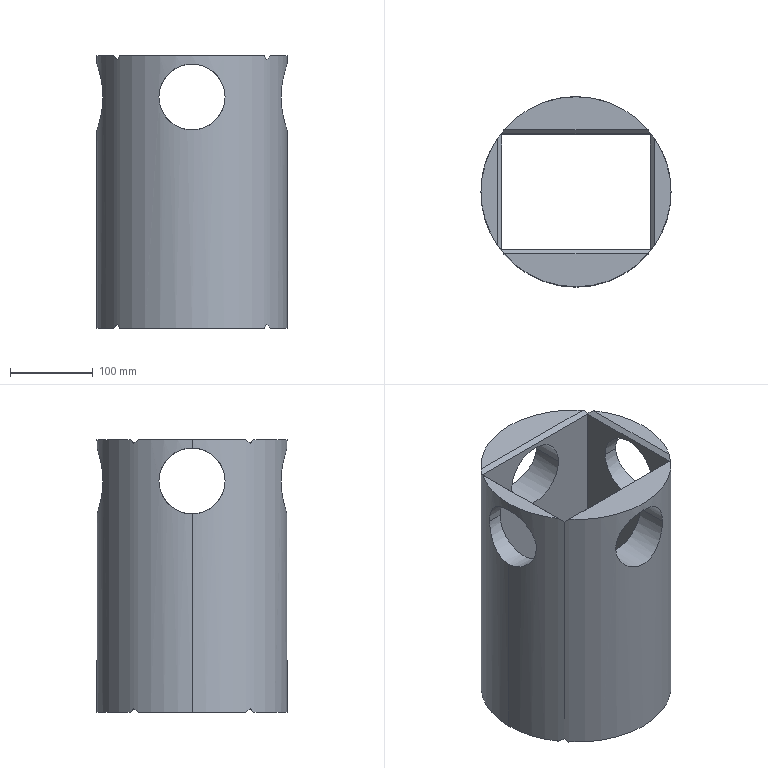Component | SolidWorks | RotatingSleeve-1 | 1 solid | 30 faces | volume 4710632 mm3 | plane 20 | cylinder 10 | commonest cylinder face diameters 80 x8 230 x2 | material 45